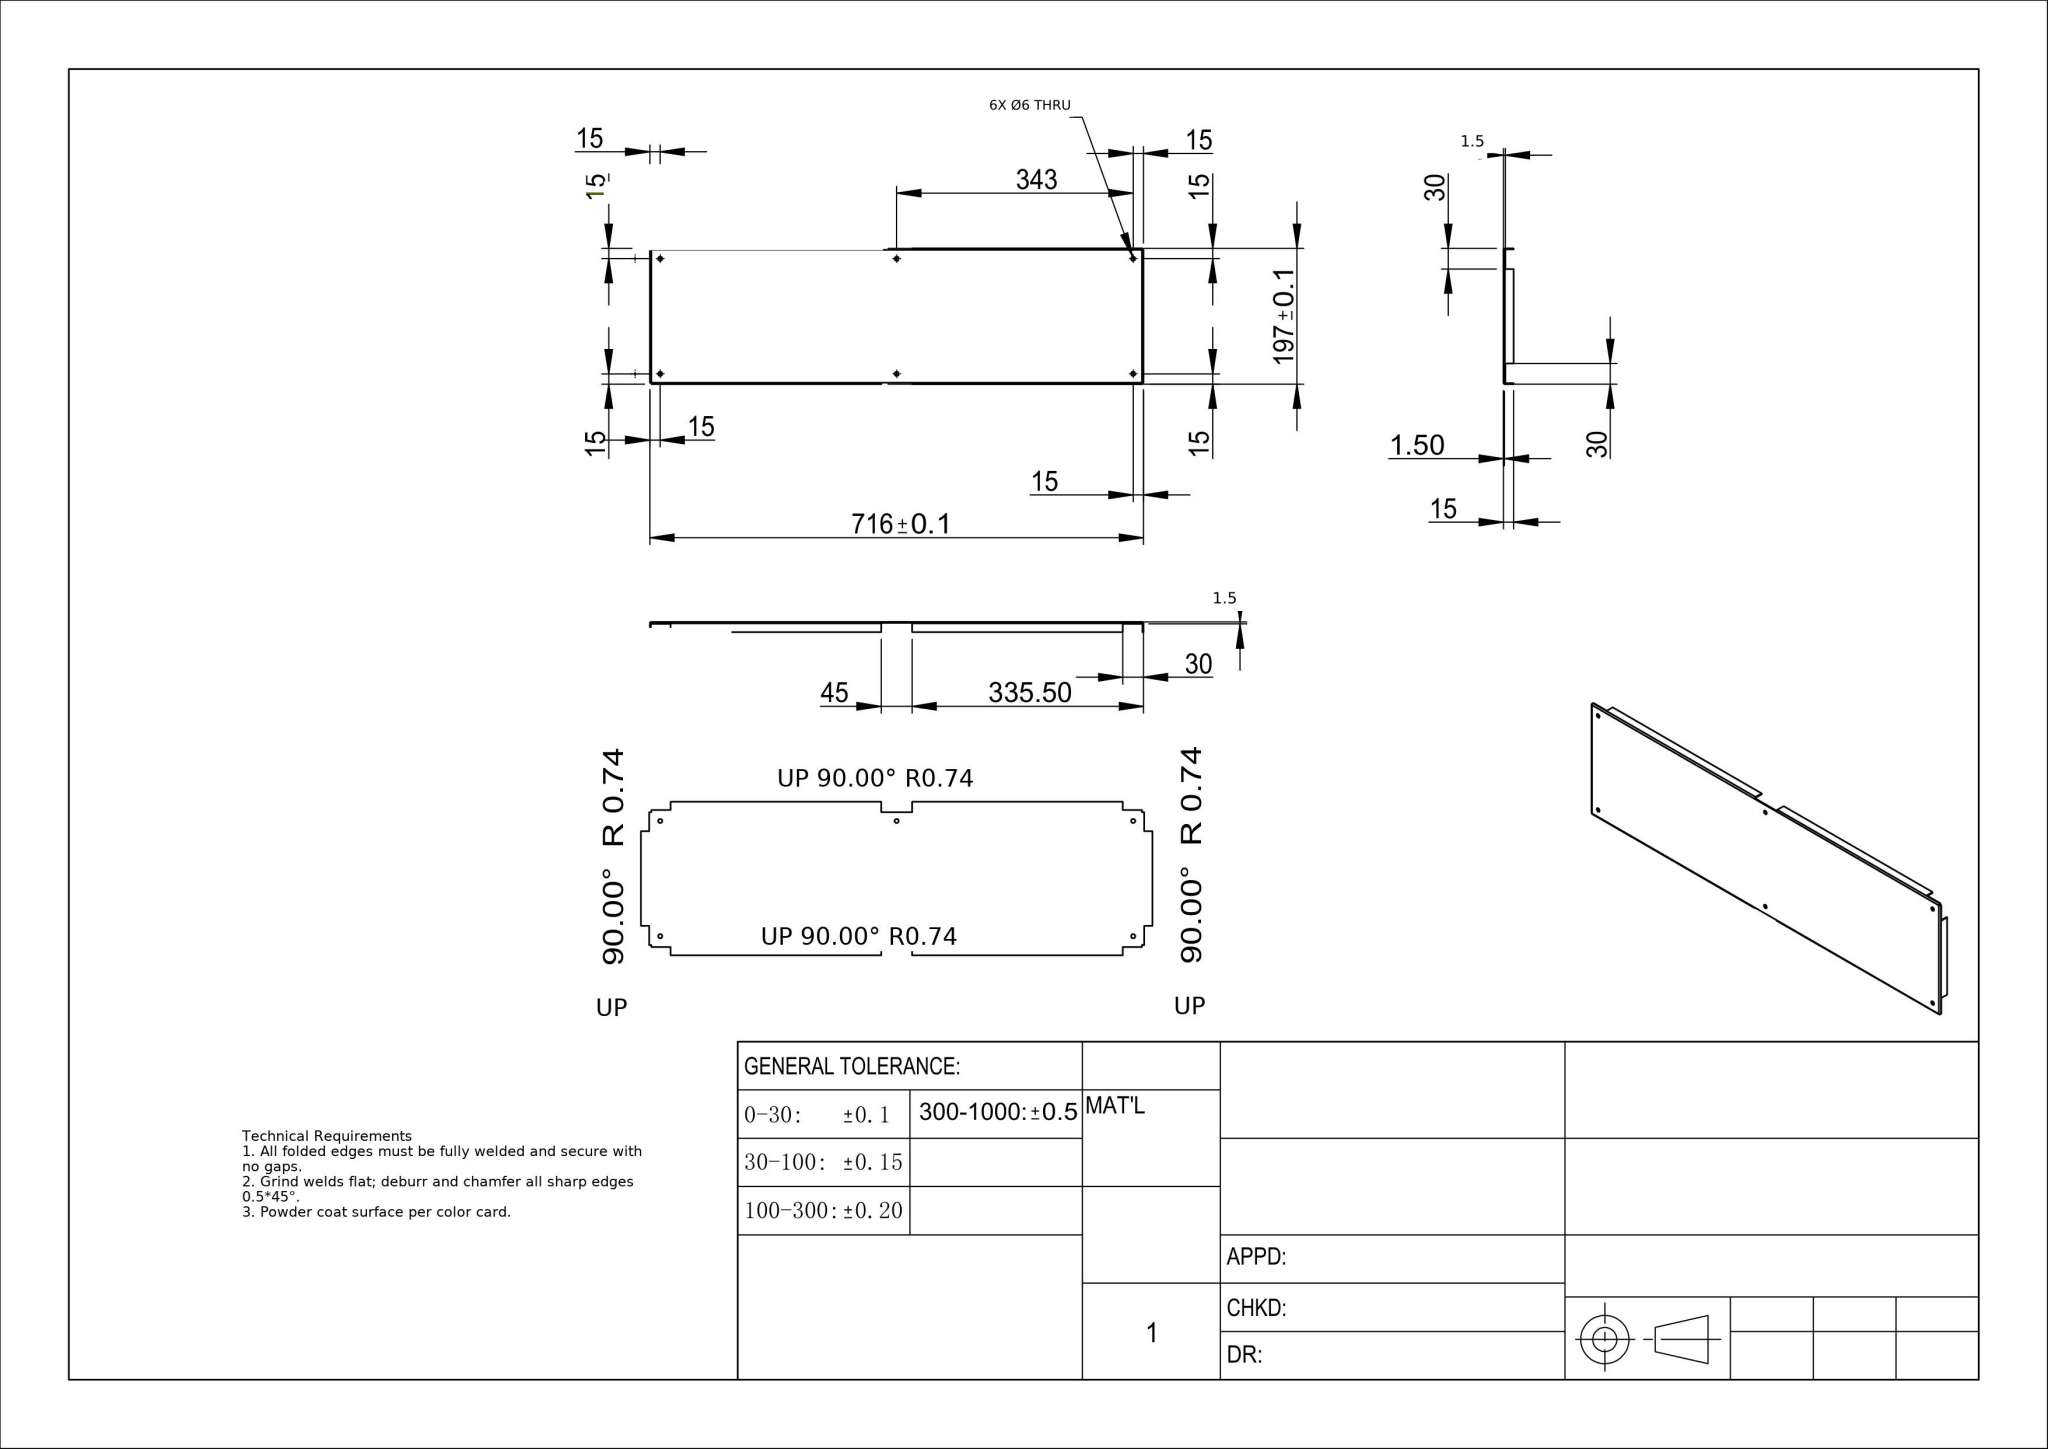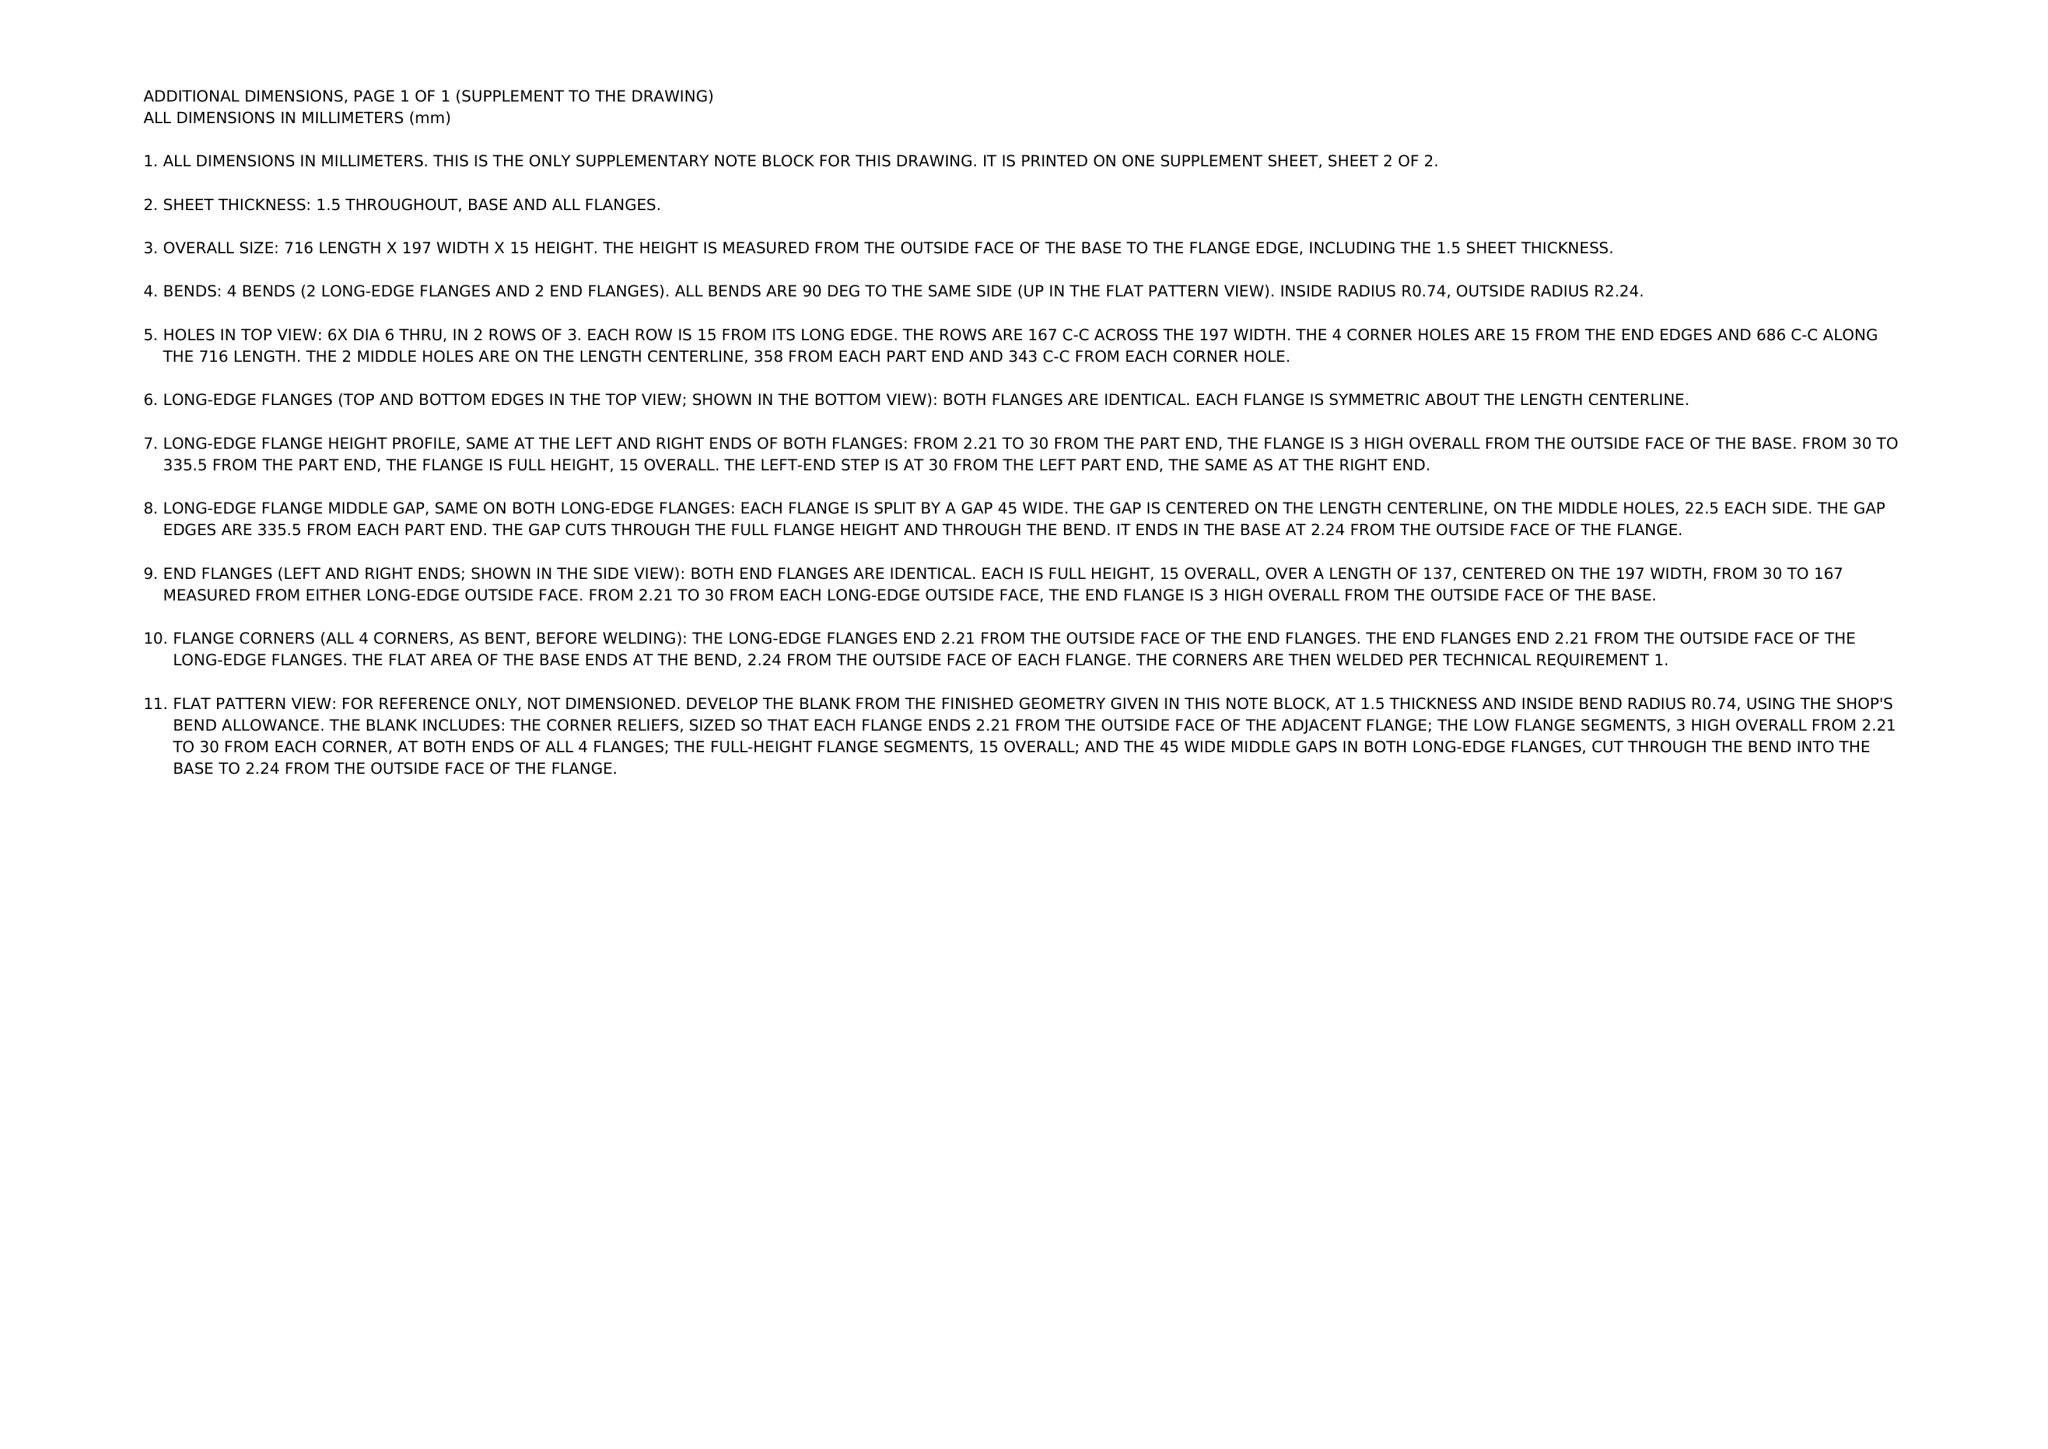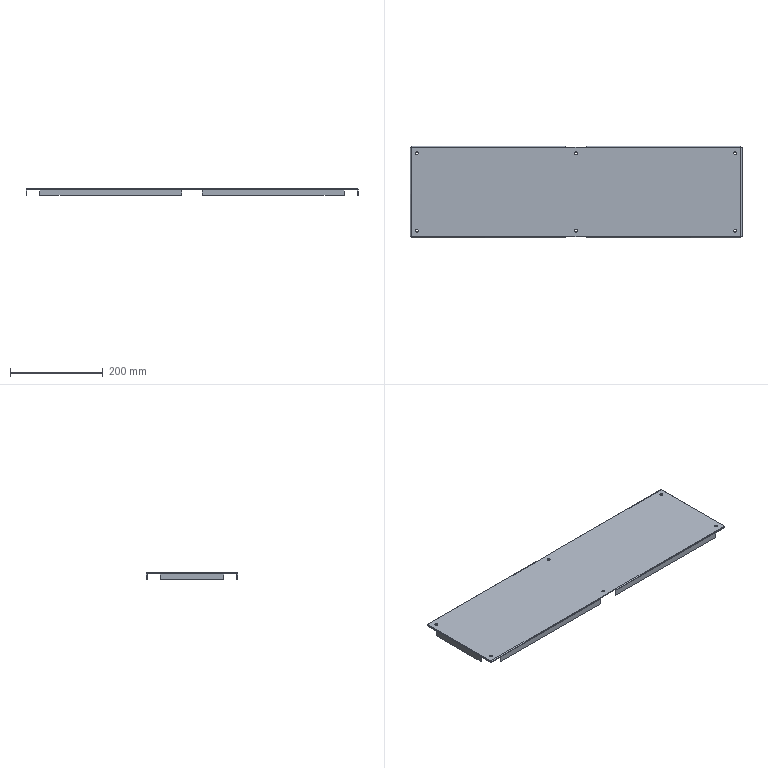Part | NX | mm | 1 solid | 86 faces | box 716 x 197 x 15 mm | volume 240142 mm3 | plane 54 | cylinder 24 | spline 8 | commonest cylinder face diameters 6 x12 4.473 x6 1.473 x6